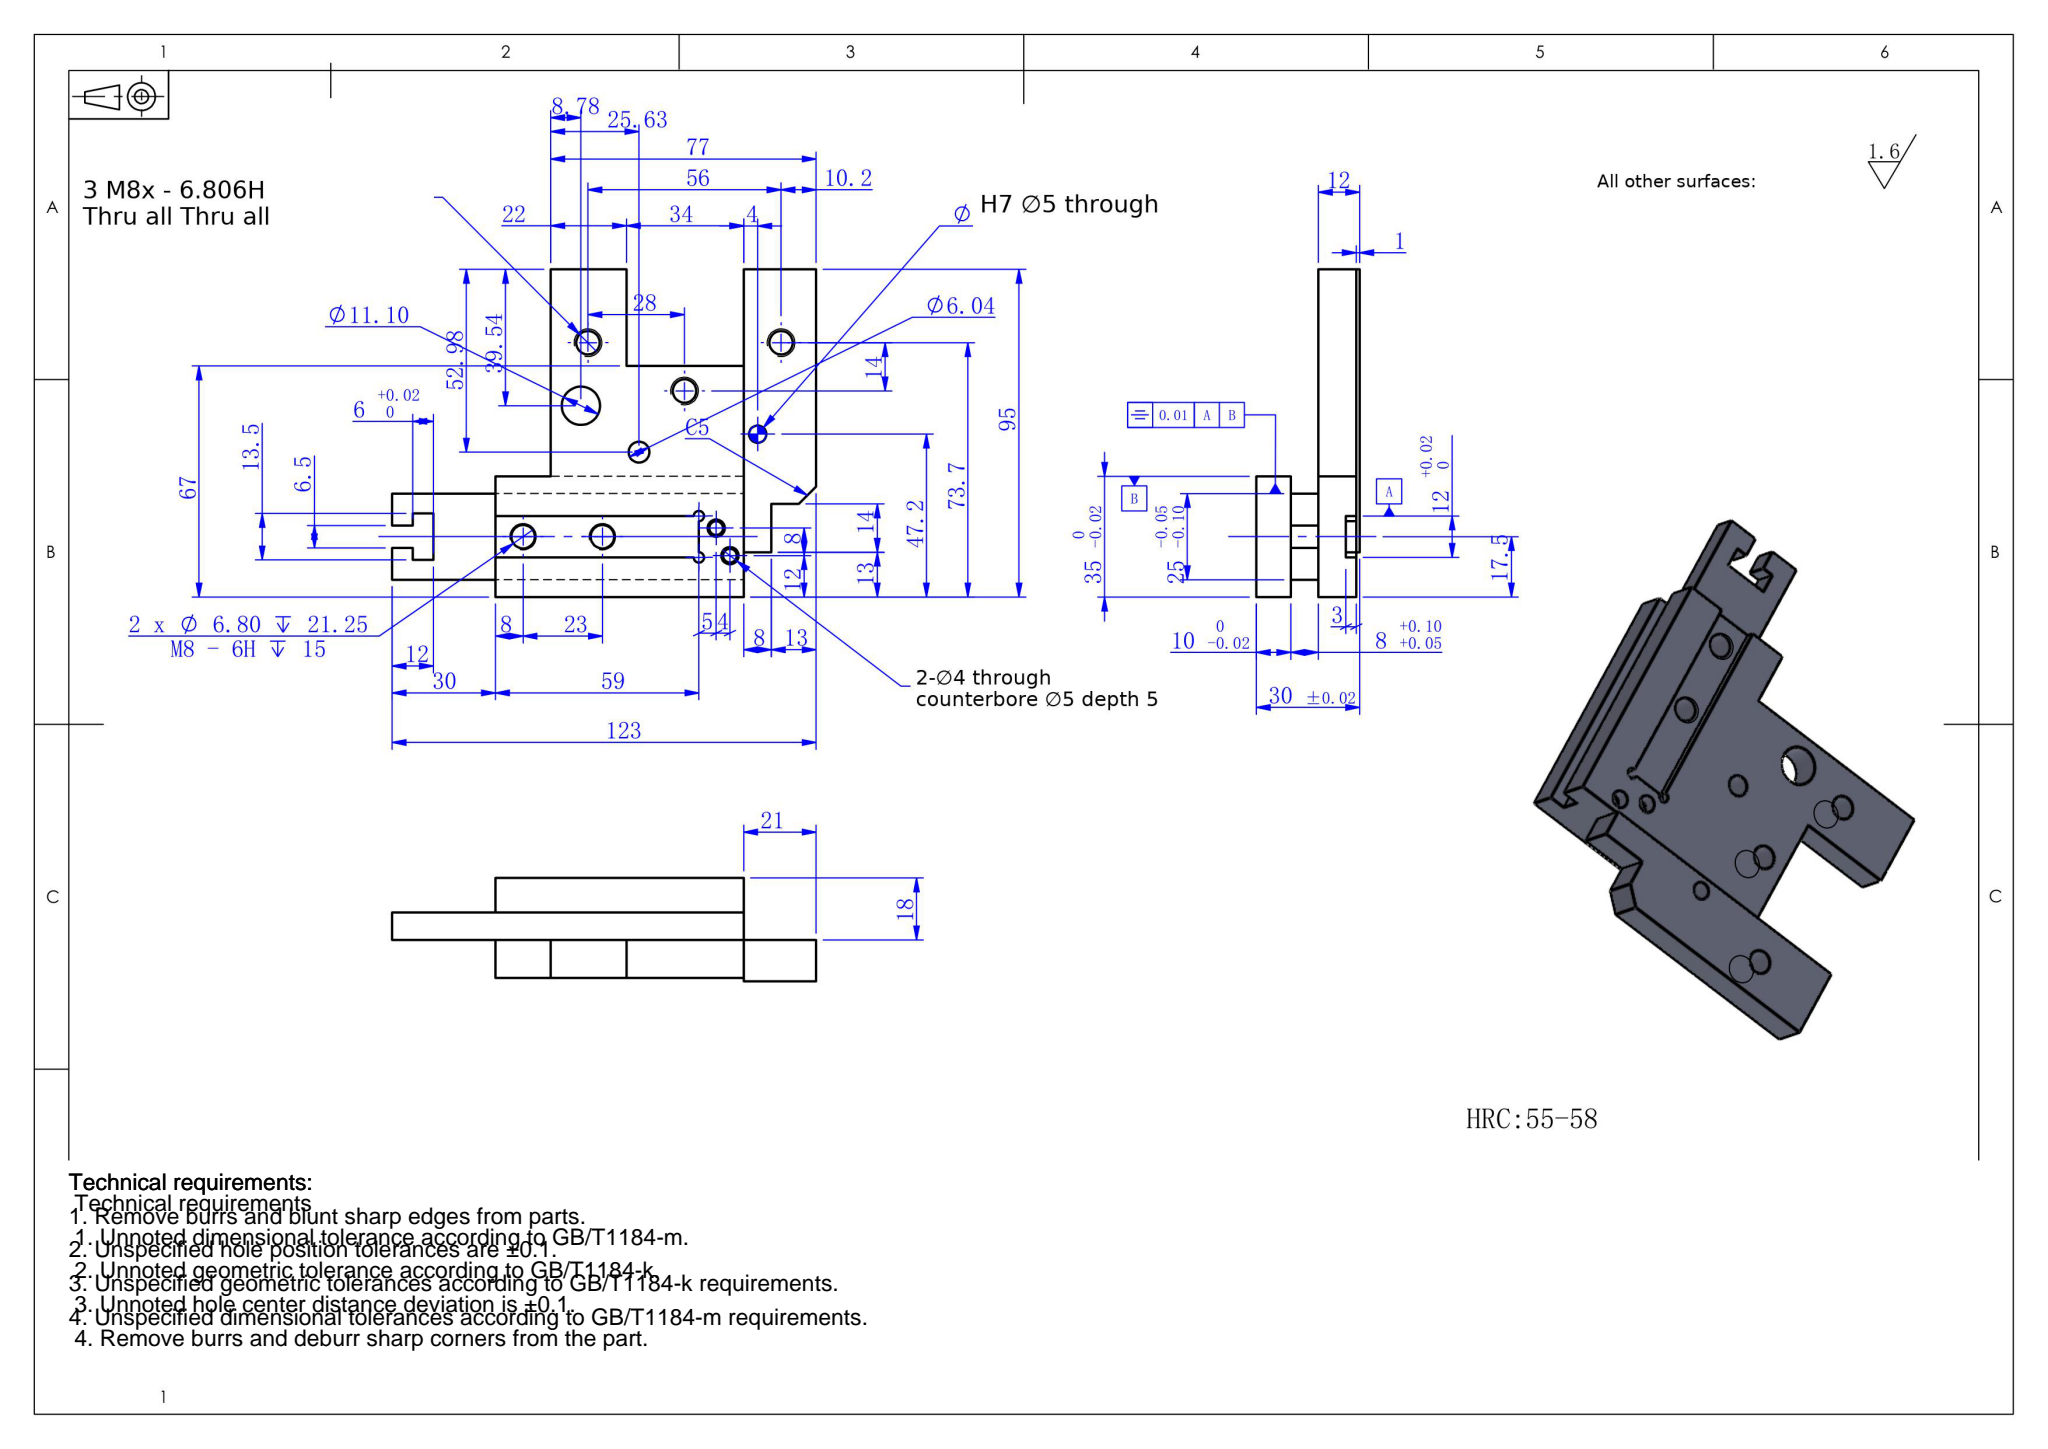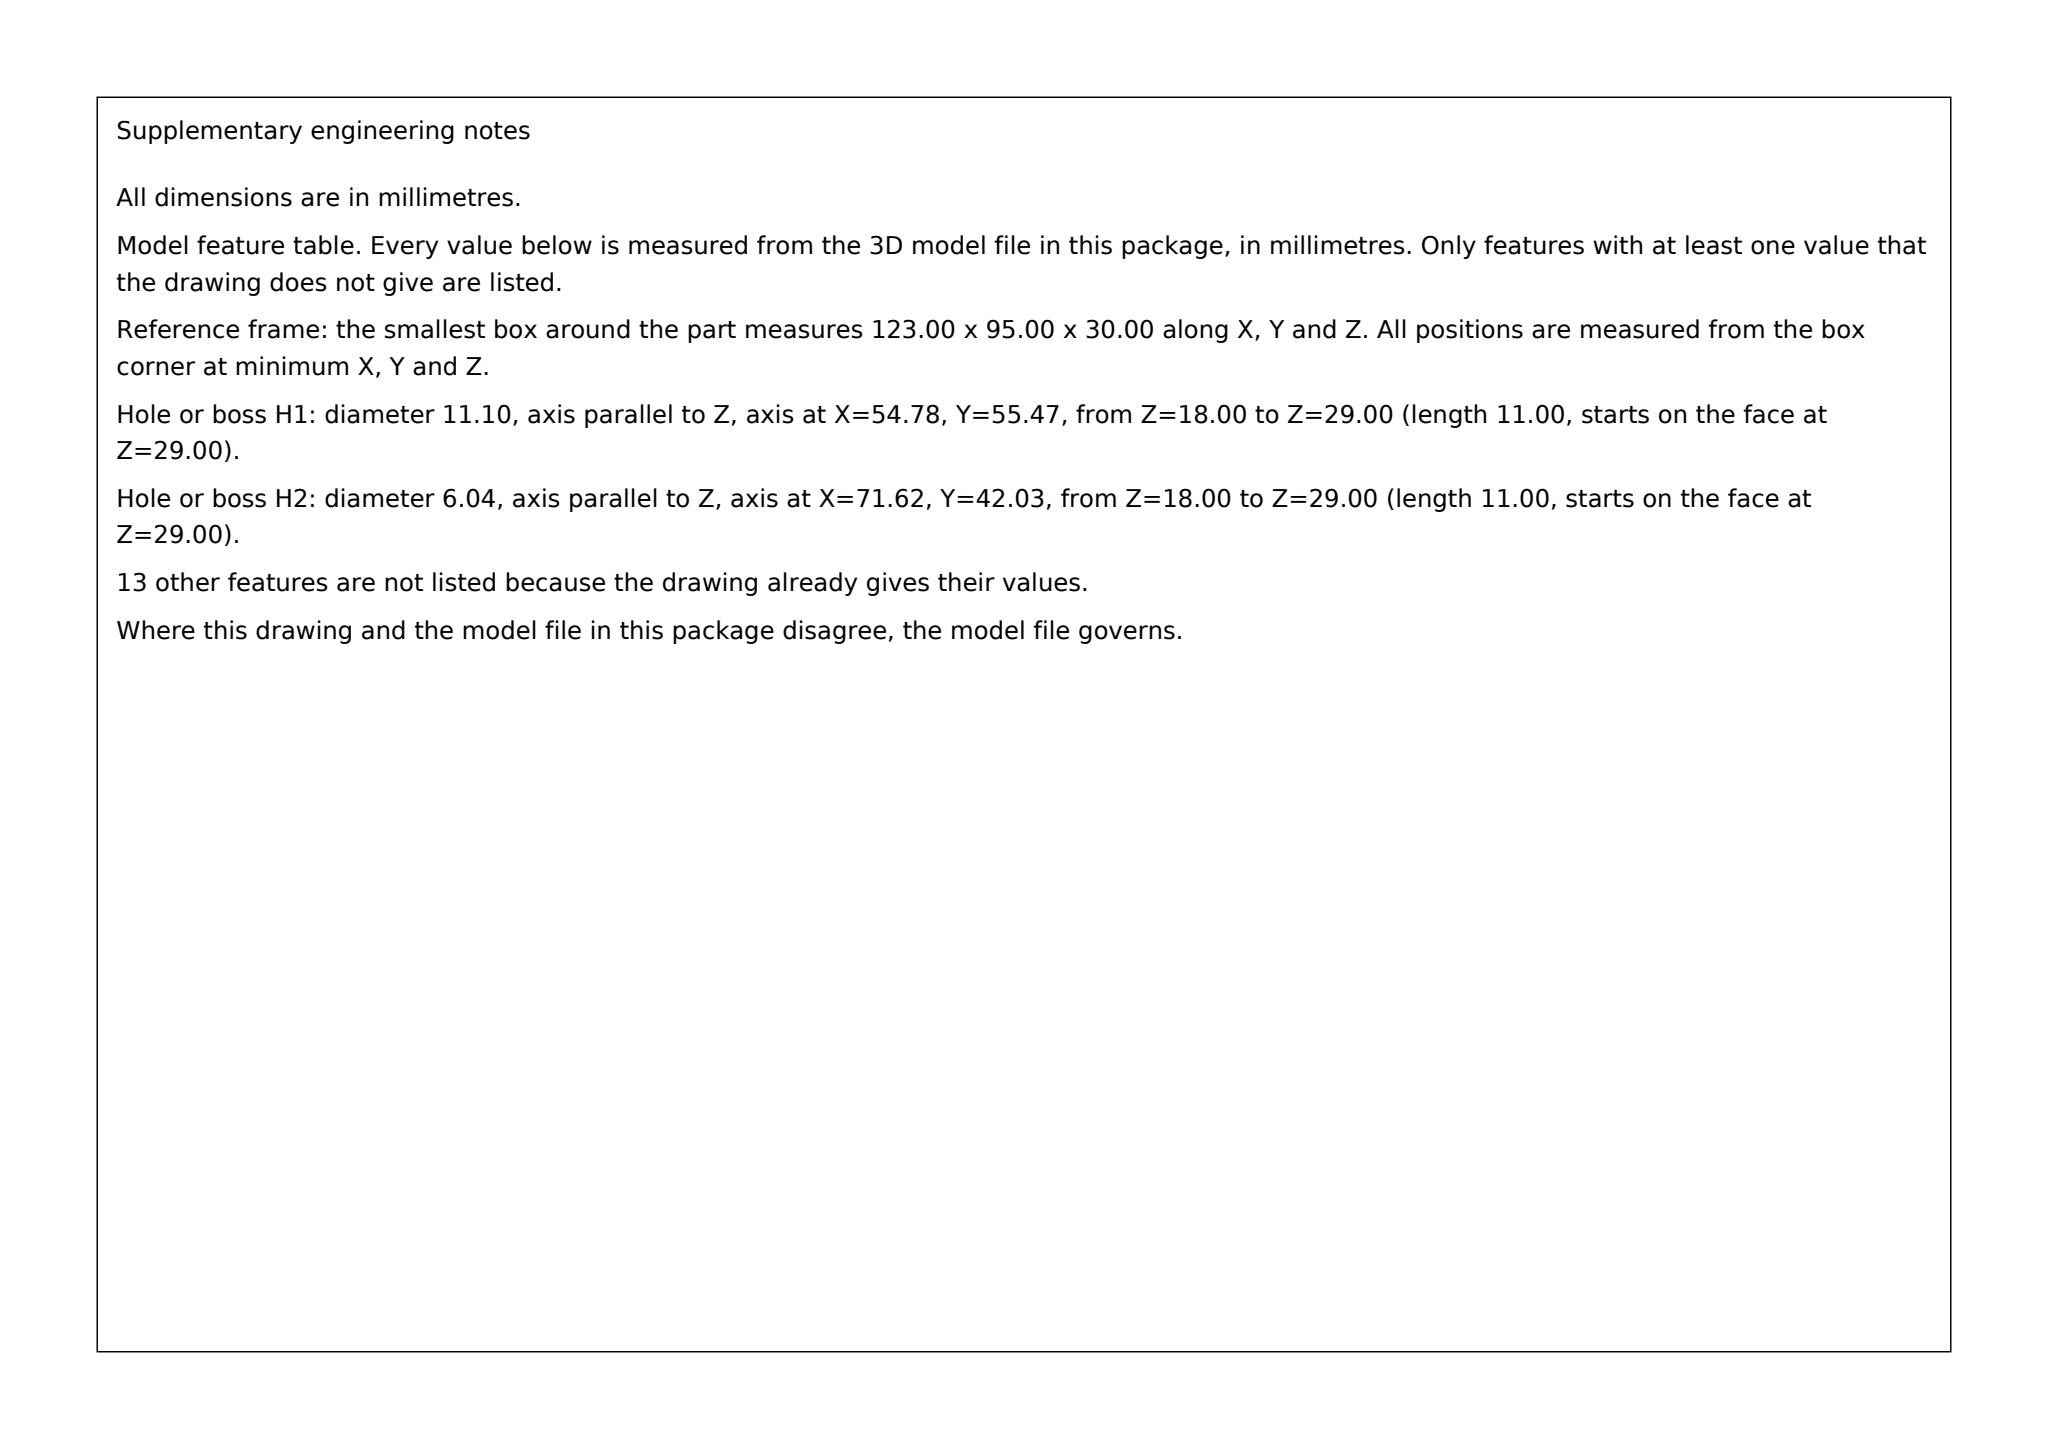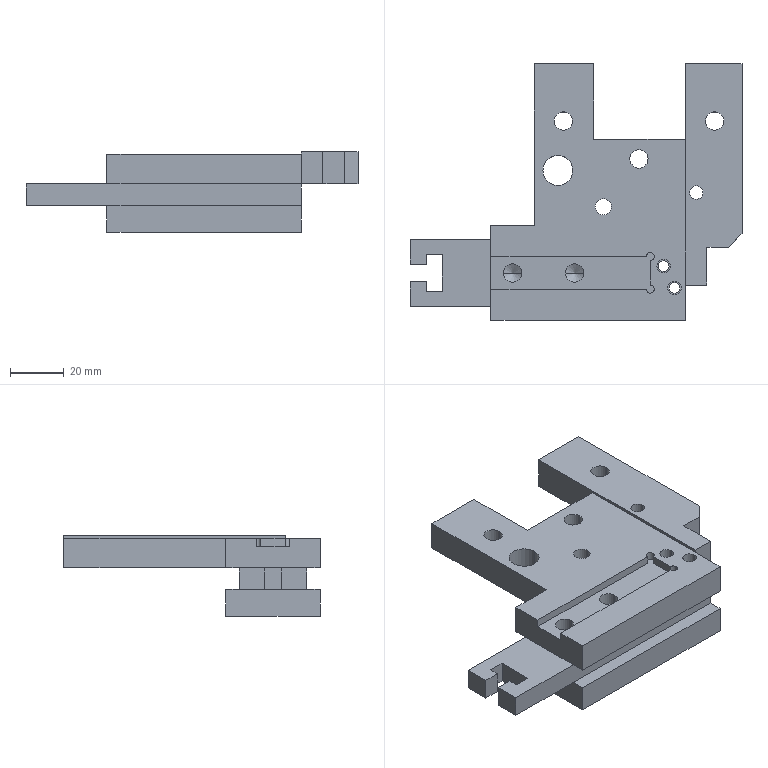Part | SolidWorks | mm | 1 solid | 76 faces | box 123 x 95 x 30 mm | volume 109779 mm3 | plane 44 | cylinder 28 | cone 4 | commonest cylinder face diameters 6.8 x10 5 x6 4 x4 3 x4 11.104 x2 6.04 x2
build123d program:
from build123d import *

# Parameters (mm, degrees)
SKETCH1_W             = 80
SKETCH1_H             = 35
BOSS_EXTRUDE1_DEPTH   = 29
SKETCH4_W             = 8
SKETCH4_H             = 5
CUT_EXTRUDE2_DEPTH    = 101.795
SKETCH5_W             = 64
SKETCH5_H             = 11
BOSS_EXTRUDE3_DEPTH   = 60
SKETCH8_W             = 8
SKETCH8_H             = 13
CUT_EXTRUDE5_DEPTH    = 50
SKETCH12_W            = 8
SKETCH12_H            = 82
BOSS_EXTRUDE5_DEPTH   = 1
SKETCH13_R            = 2.5
CUT_EXTRUDE6_DEPTH    = 157.685
SKETCH14_W            = 12
SKETCH14_H            = 68
BOSS_EXTRUDE6_DEPTH   = 13
CHAMFER1_SIZE         = 5
SKETCH15_W            = 34
SKETCH15_H            = 28
CUT_EXTRUDE7_DEPTH    = 157.496
SKETCH16_W            = 3
SKETCH16_H            = 12
CUT_EXTRUDE8_DEPTH    = 59
SKETCH17_R            = 1.5
CUT_EXTRUDE9_DEPTH    = 3
M8_TAPPED_HOLE2_D     = 6.8
SKETCH22_R            = 2.5
CUT_EXTRUDE10_DEPTH   = 5
SKETCH23_R            = 2
CUT_EXTRUDE11_DEPTH   = 156.647
SKETCH24_W            = 8
SKETCH24_H            = 25
BOSS_EXTRUDE7_DEPTH   = 30
SKETCH25_W            = 6
SKETCH25_H            = 13.5
CUT_EXTRUDE12_DEPTH   = 177.254
SKETCH26_W            = 6
SKETCH26_H            = 6.5
CUT_EXTRUDE13_DEPTH   = 10
SKETCH27_W            = 18
SKETCH27_H            = 30
CUT_EXTRUDE14_DEPTH   = 8
M8_TAPPED_HOLE3_D     = 6.8
M8_TAPPED_HOLE3_DEPTH = 21.25
M8_TAPPED_HOLE3_TIP   = 2.043
SKETCH30_R            = 5.552
SKETCH30_R_2          = 3.02
CUT_EXTRUDE15_DEPTH   = 51


with BuildPart() as part:
    # Sketch1 → Boss-Extrude1 (new body)
    with BuildSketch(Plane.XY):
        with Locations((-63.192, 36.525)):
            Rectangle(SKETCH1_W, SKETCH1_H)
    extrude(amount=BOSS_EXTRUDE1_DEPTH)

    # Sketch4 → Cut-Extrude2 (cut, through all)
    with BuildSketch(Plane.ZY.offset(103.192)):
        with Locations((14, 51.525)):
            Rectangle(SKETCH4_W, SKETCH4_H)
        with Locations((14, 21.525)):
            Rectangle(SKETCH4_W, SKETCH4_H)
    extrude(amount=-CUT_EXTRUDE2_DEPTH, mode=Mode.SUBTRACT)

    # Sketch5 → Boss-Extrude3 (add)
    with BuildSketch(Plane(origin=(0, 54.025, 0), x_dir=(1, 0, 0), z_dir=(0, 1, 0))):
        with Locations((-55.192, -23.5)):
            Rectangle(SKETCH5_W, SKETCH5_H)
    extrude(amount=BOSS_EXTRUDE3_DEPTH)

    # Sketch8 → Cut-Extrude5 (cut)
    with BuildSketch(Plane(origin=(0, 0, 0), x_dir=(-1, 0, 0), z_dir=(0, 0, -1))):
        with Locations((27.192, 25.525)):
            Rectangle(SKETCH8_W, SKETCH8_H)
    extrude(amount=-CUT_EXTRUDE5_DEPTH, mode=Mode.SUBTRACT)

    # Sketch12 → Boss-Extrude5 (add)
    with BuildSketch(Plane.XY.offset(29)):
        with Locations((-27.192, 73.025)):
            Rectangle(SKETCH12_W, SKETCH12_H)
    extrude(amount=BOSS_EXTRUDE5_DEPTH)

    # Sketch13 → Cut-Extrude6 (cut, through all)
    with BuildSketch(Plane.XY.offset(30)):
        with Locations((-27.143, 66.264)):
            Circle(SKETCH13_R)
    extrude(amount=-CUT_EXTRUDE6_DEPTH, mode=Mode.SUBTRACT)

    # Sketch14 → Boss-Extrude6 (add)
    with BuildSketch(Plane(origin=(-23.192, 0, 0), x_dir=(0, 0, -1), z_dir=(1, 0, 0))):
        with Locations((-24, 80.025)):
            Rectangle(SKETCH14_W, SKETCH14_H)
    extrude(amount=BOSS_EXTRUDE6_DEPTH)

    # Chamfer1
    chamfer1_edges = [part.edges().sort_by_distance(p)[0] for p in [
        (-10.192, 46.025, 24),
    ]]
    chamfer(chamfer1_edges, length=CHAMFER1_SIZE)

    # Sketch15 → Cut-Extrude7 (cut, through all)
    with BuildSketch(Plane.XY.offset(29)):
        with Locations((-48.192, 100.025)):
            Rectangle(SKETCH15_W, SKETCH15_H)
    extrude(amount=-CUT_EXTRUDE7_DEPTH, mode=Mode.SUBTRACT)

    # Sketch16 → Cut-Extrude8 (cut)
    with BuildSketch(Plane.ZY.offset(103.192)):
        with Locations((27.5, 36.525)):
            Rectangle(SKETCH16_W, SKETCH16_H)
    extrude(amount=-CUT_EXTRUDE8_DEPTH, mode=Mode.SUBTRACT)

    # Sketch17 → Cut-Extrude9 (cut)
    with BuildSketch(Plane.XY.offset(29)):
        with Locations((-44.192, 42.525)):
            Circle(SKETCH17_R)
        with Locations((-44.192, 30.525)):
            Circle(SKETCH17_R)
    extrude(amount=-CUT_EXTRUDE9_DEPTH, mode=Mode.SUBTRACT)

    # M8 Tapped Hole2 (through all)
    with Locations(Plane(origin=(0, 0, 18), x_dir=(-1, 0, 0), z_dir=(0, 0, -1))):
        with Locations((20.37, 92.764), (48.37, 78.764), (76.37, 92.764)):
            Hole(M8_TAPPED_HOLE2_D / 2)

    # Sketch22 → Cut-Extrude10 (cut)
    with BuildSketch(Plane.XY.offset(29)):
        with Locations((-39.192, 39.025)):
            Circle(SKETCH22_R)
        with Locations((-35.192, 31.025)):
            Circle(SKETCH22_R)
    extrude(amount=-CUT_EXTRUDE10_DEPTH, mode=Mode.SUBTRACT)

    # Sketch23 → Cut-Extrude11 (cut, through all)
    with BuildSketch(Plane.XY.offset(24)):
        with Locations((-39.192, 39.025)):
            Circle(SKETCH23_R)
        with Locations((-35.192, 31.025)):
            Circle(SKETCH23_R)
    extrude(amount=-CUT_EXTRUDE11_DEPTH, mode=Mode.SUBTRACT)

    # Sketch24 → Boss-Extrude7 (add)
    with BuildSketch(Plane.ZY.offset(103.192)):
        with Locations((14, 36.525)):
            Rectangle(SKETCH24_W, SKETCH24_H)
    extrude(amount=BOSS_EXTRUDE7_DEPTH)

    # Sketch25 → Cut-Extrude12 (cut, through all)
    with BuildSketch(Plane.XY.offset(18)):
        with Locations((-124.192, 36.525)):
            Rectangle(SKETCH25_W, SKETCH25_H)
    extrude(amount=-CUT_EXTRUDE12_DEPTH, mode=Mode.SUBTRACT)

    # Sketch26 → Cut-Extrude13 (cut)
    with BuildSketch(Plane.XY.offset(18)):
        with Locations((-130.192, 36.525)):
            Rectangle(SKETCH26_W, SKETCH26_H)
    extrude(amount=-CUT_EXTRUDE13_DEPTH, mode=Mode.SUBTRACT)

    # Sketch27 → Cut-Extrude14 (cut)
    with BuildSketch(Plane(origin=(-23.192, 0, 0), x_dir=(0, 0, -1), z_dir=(1, 0, 0))):
        with Locations((-9, 39.025)):
            Rectangle(SKETCH27_W, SKETCH27_H)
    extrude(amount=-CUT_EXTRUDE14_DEPTH, mode=Mode.SUBTRACT)

    # M8 Tapped Hole3
    with Locations(Plane.XY.offset(26)):
        with Locations((-95.192, 36.525), (-72.192, 36.525)):
            Hole(M8_TAPPED_HOLE3_D / 2, depth=M8_TAPPED_HOLE3_DEPTH)
            with Locations((0, 0, -(M8_TAPPED_HOLE3_DEPTH + M8_TAPPED_HOLE3_TIP / 2))):  # 118° drill point
                Cone(0, M8_TAPPED_HOLE3_D / 2, M8_TAPPED_HOLE3_TIP, mode=Mode.SUBTRACT)

    # Sketch30 → Cut-Extrude15 (cut)
    with BuildSketch(Plane.XY.offset(29)):
        with Locations((-78.412, 74.488)):
            Circle(SKETCH30_R)
        with Locations((-61.565, 61.047)):
            Circle(SKETCH30_R_2)
    extrude(amount=-CUT_EXTRUDE15_DEPTH, mode=Mode.SUBTRACT)


solid = part.part